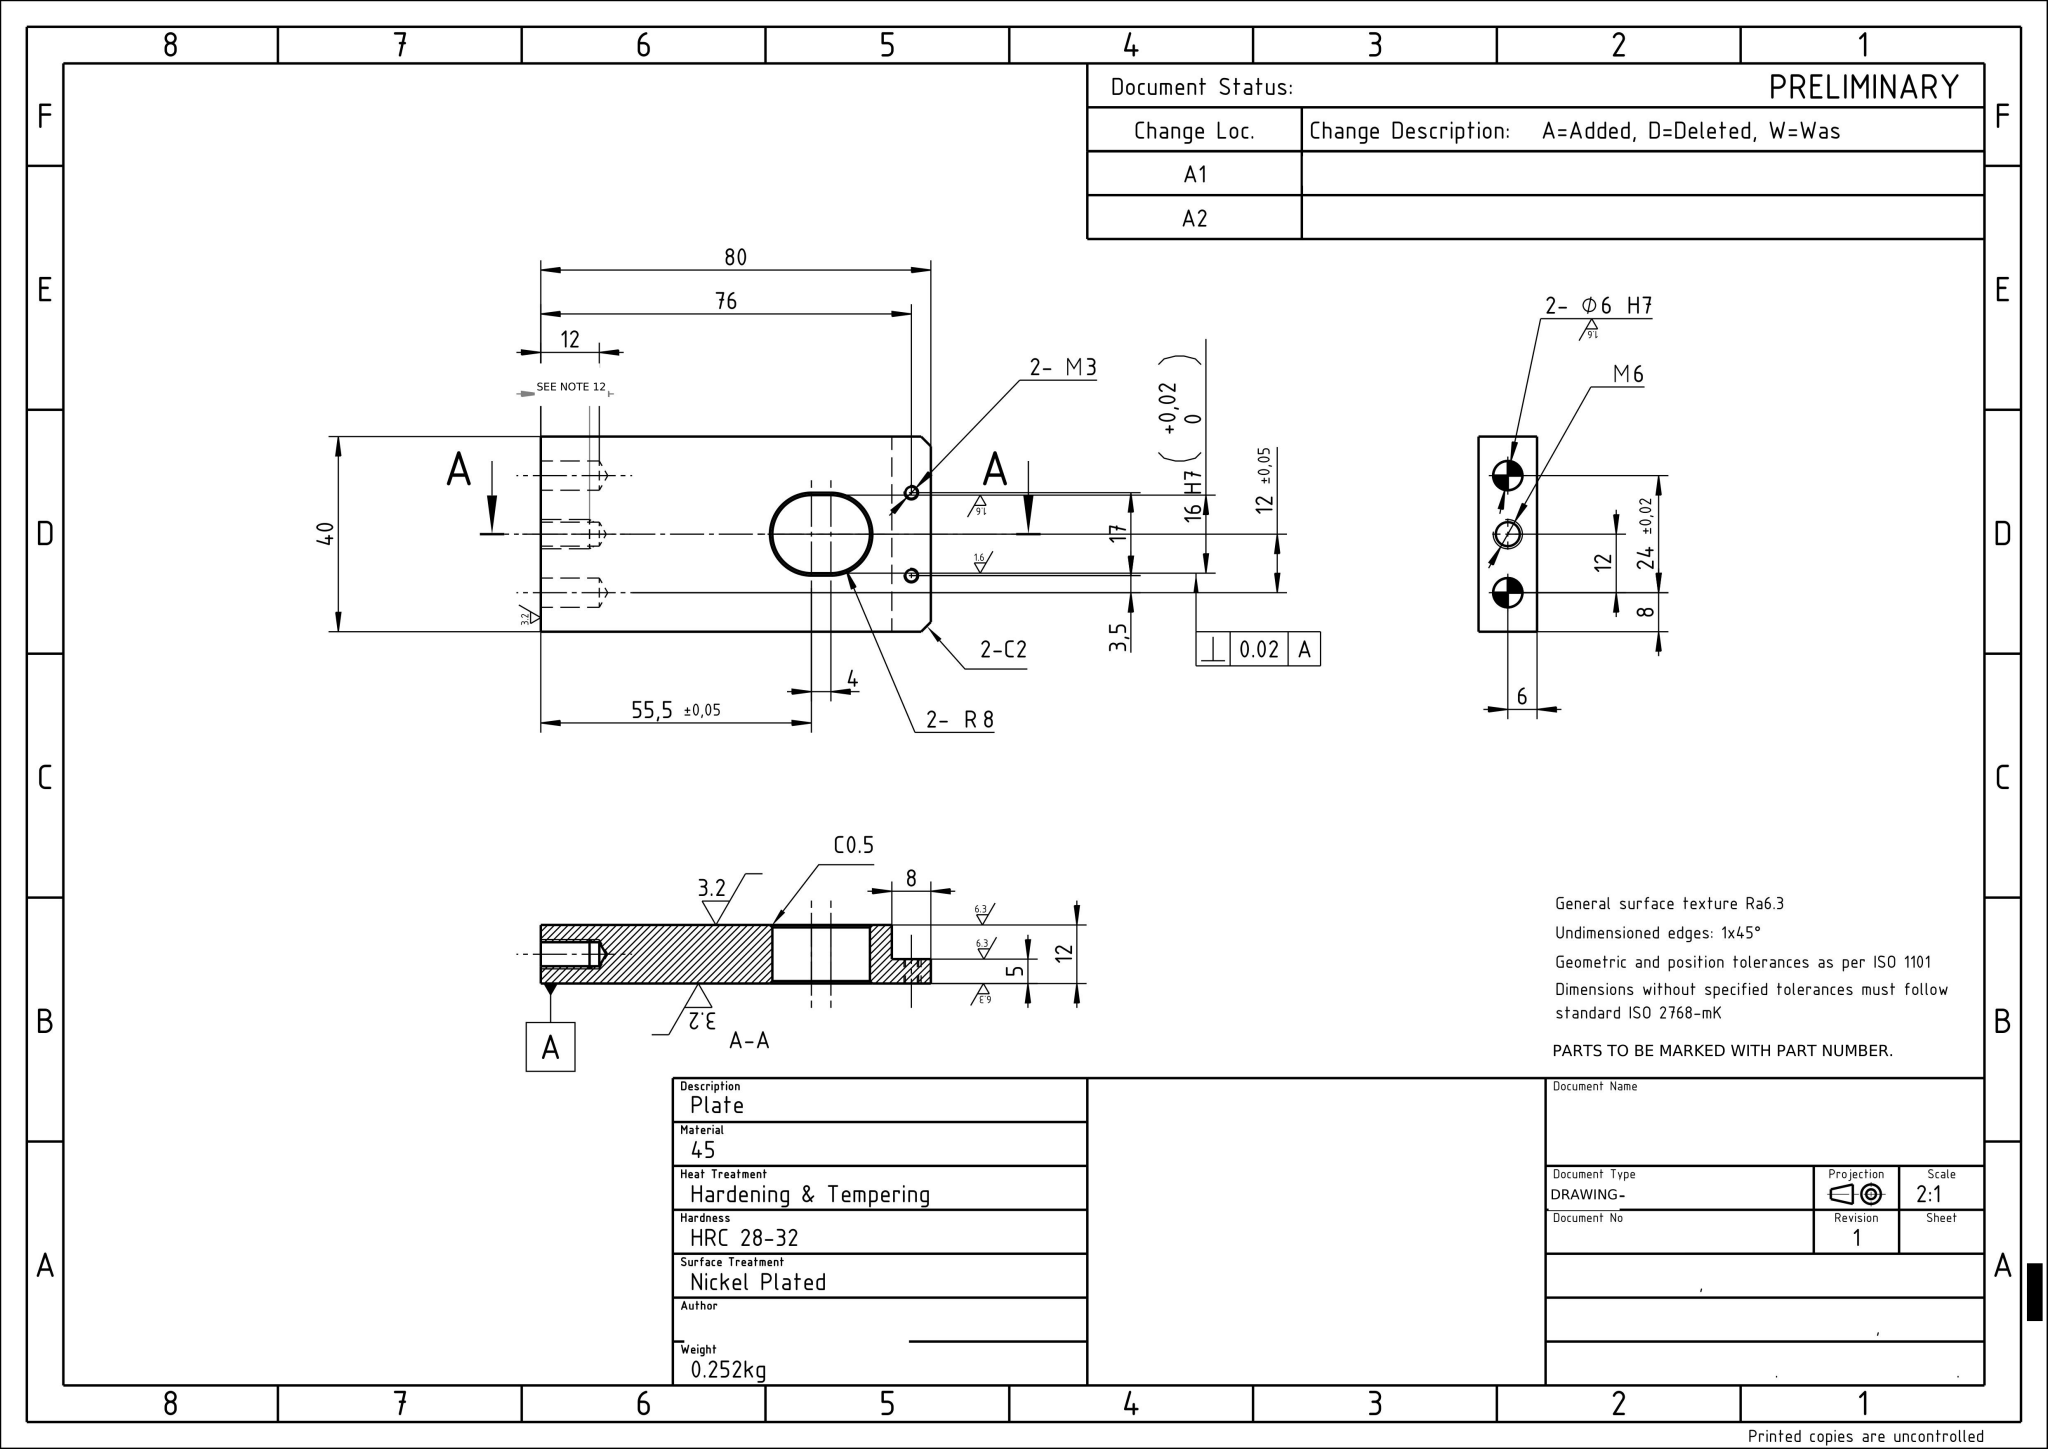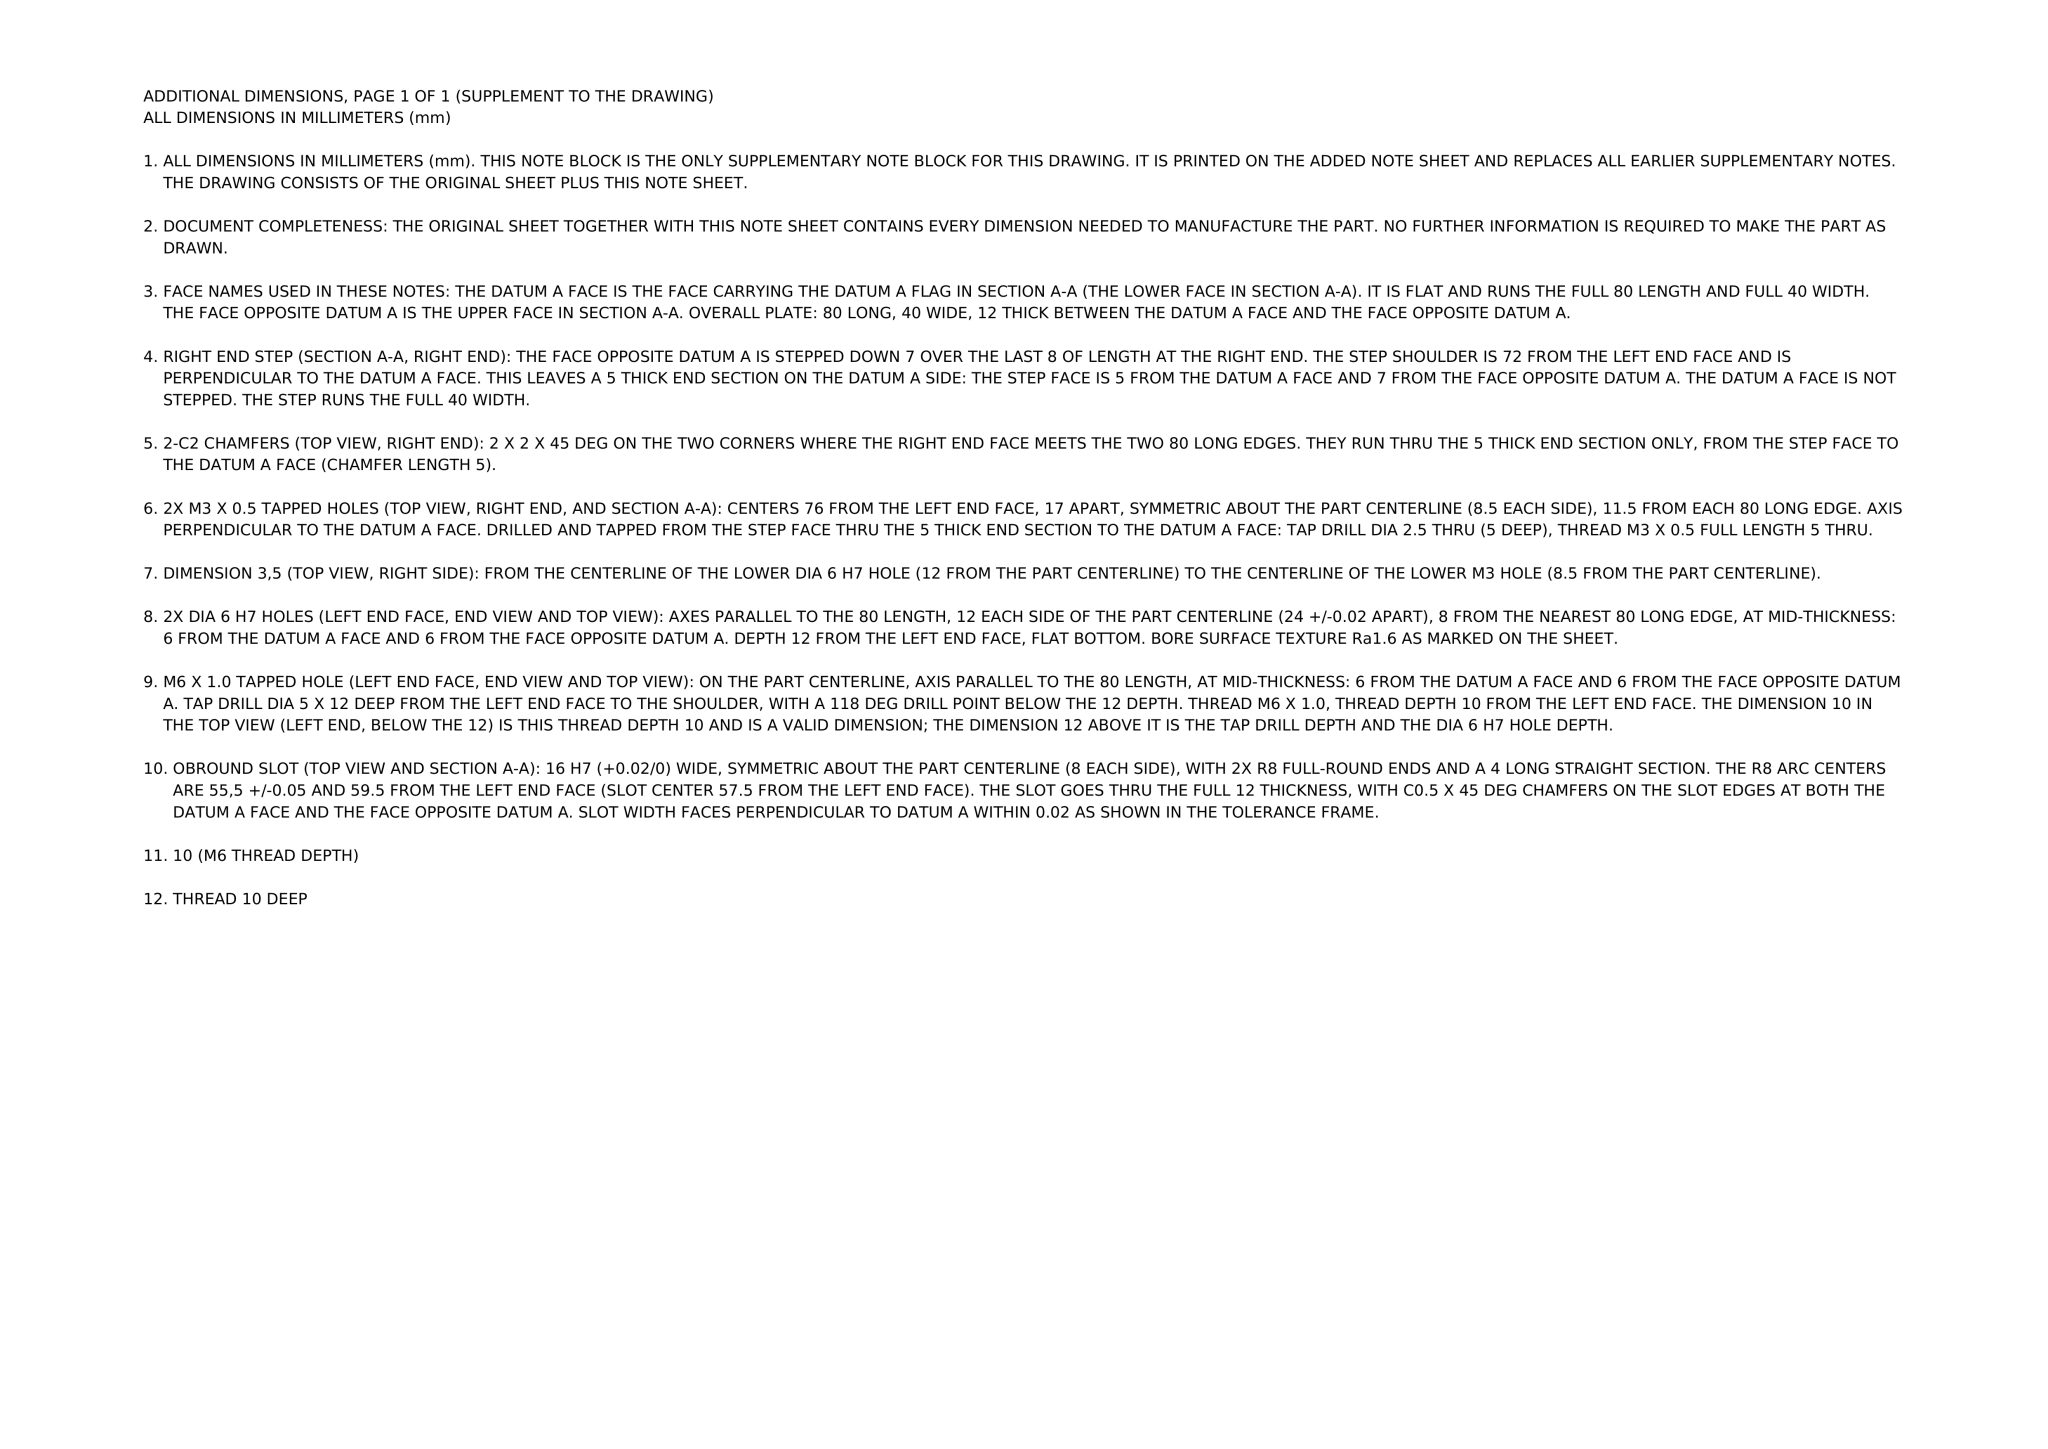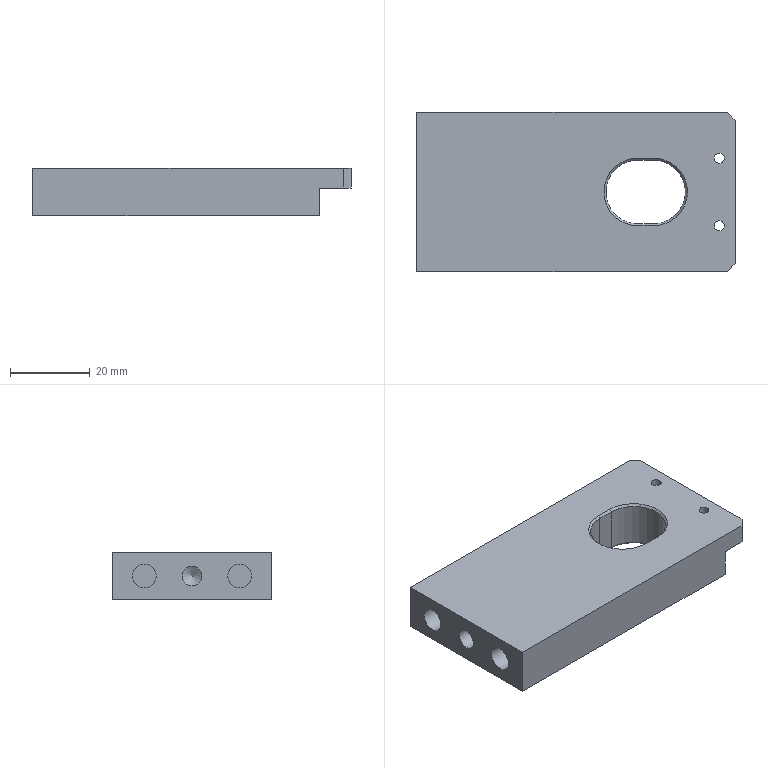Part | NX | mm | 1 solid | 30 faces | box 80 x 40 x 12 mm | volume 31971 mm3 | plane 18 | cylinder 7 | cone 5 | commonest cylinder face diameters 16 x2 2.5 x2 6 x2 5 x1
STEP:
#1=CARTESIAN_POINT('',(0.,0.,0.));
#2=DIRECTION('',(0.,0.,1.));
#3=DIRECTION('',(1.,0.,0.));
#4=AXIS2_PLACEMENT_3D('',#1,#2,#3);
#5=(LENGTH_UNIT()NAMED_UNIT(*)SI_UNIT(.MILLI.,.METRE.));
#6=UNCERTAINTY_MEASURE_WITH_UNIT(LENGTH_MEASURE(0.00002),#5,'','');
#7=(NAMED_UNIT(*)PLANE_ANGLE_UNIT()SI_UNIT($,.RADIAN.));
#8=PLANE_ANGLE_MEASURE_WITH_UNIT(PLANE_ANGLE_MEASURE(0.01745),#7);
#9=DIMENSIONAL_EXPONENTS(0.,0.,0.,0.,0.,0.,0.);
#10=(CONVERSION_BASED_UNIT('',#8)NAMED_UNIT(#9)PLANE_ANGLE_UNIT());
#11=(NAMED_UNIT(*)SI_UNIT($,.STERADIAN.)SOLID_ANGLE_UNIT());
#12=(GEOMETRIC_REPRESENTATION_CONTEXT(3)GLOBAL_UNCERTAINTY_ASSIGNED_CONTEXT((#6))GLOBAL_UNIT_ASSIGNED_CONTEXT((#5,#10,#11))REPRESENTATION_CONTEXT('',''));
#13=SHAPE_REPRESENTATION('',(#4),#12);
#14=CARTESIAN_POINT('',(34.75,8.5,12.));
#15=VERTEX_POINT('',#14);
#16=CARTESIAN_POINT('',(36.,8.5,12.));
#17=DIRECTION('',(0.,0.,-1.));
#18=DIRECTION('',(-1.,0.,0.));
#19=AXIS2_PLACEMENT_3D('',#16,#17,#18);
#20=CIRCLE('',#19,1.25);
#21=EDGE_CURVE('',#15,#15,#20,.T.);
#22=ORIENTED_EDGE('',*,*,#21,.T.);
#23=EDGE_LOOP('',(#22));
#24=FACE_BOUND('',#23,.T.);
#25=CARTESIAN_POINT('',(34.75,-8.5,12.));
#26=VERTEX_POINT('',#25);
#27=CARTESIAN_POINT('',(36.,-8.5,12.));
#28=DIRECTION('',(0.,0.,-1.));
#29=DIRECTION('',(-1.,0.,0.));
#30=AXIS2_PLACEMENT_3D('',#27,#28,#29);
#31=CIRCLE('',#30,1.25);
#32=EDGE_CURVE('',#26,#26,#31,.T.);
#33=ORIENTED_EDGE('',*,*,#32,.T.);
#34=EDGE_LOOP('',(#33));
#35=FACE_BOUND('',#34,.T.);
#36=CARTESIAN_POINT('',(19.5,-8.5,12.));
#37=VERTEX_POINT('',#36);
#38=CARTESIAN_POINT('',(15.5,-8.5,12.));
#39=VERTEX_POINT('',#38);
#40=CARTESIAN_POINT('',(0.,-8.5,12.));
#41=DIRECTION('',(-1.,0.,0.));
#42=VECTOR('',#41,1.);
#43=LINE('',#40,#42);
#44=EDGE_CURVE('',#37,#39,#43,.T.);
#45=ORIENTED_EDGE('',*,*,#44,.T.);
#46=CARTESIAN_POINT('',(15.5,8.5,12.));
#47=VERTEX_POINT('',#46);
#48=CARTESIAN_POINT('',(15.5,0.,12.));
#49=DIRECTION('',(0.,0.,-1.));
#50=DIRECTION('',(1.,0.,0.));
#51=AXIS2_PLACEMENT_3D('',#48,#49,#50);
#52=CIRCLE('',#51,8.5);
#53=EDGE_CURVE('',#39,#47,#52,.T.);
#54=ORIENTED_EDGE('',*,*,#53,.T.);
#55=CARTESIAN_POINT('',(19.5,8.5,12.));
#56=VERTEX_POINT('',#55);
#57=CARTESIAN_POINT('',(0.,8.5,12.));
#58=DIRECTION('',(1.,0.,0.));
#59=VECTOR('',#58,1.);
#60=LINE('',#57,#59);
#61=EDGE_CURVE('',#47,#56,#60,.T.);
#62=ORIENTED_EDGE('',*,*,#61,.T.);
#63=CARTESIAN_POINT('',(19.5,-0.,12.));
#64=DIRECTION('',(0.,0.,-1.));
#65=DIRECTION('',(1.,0.,0.));
#66=AXIS2_PLACEMENT_3D('',#63,#64,#65);
#67=CIRCLE('',#66,8.5);
#68=EDGE_CURVE('',#56,#37,#67,.T.);
#69=ORIENTED_EDGE('',*,*,#68,.T.);
#70=EDGE_LOOP('',(#45,#54,#62,#69));
#71=FACE_BOUND('',#70,.T.);
#72=CARTESIAN_POINT('',(40.,-18.,12.));
#73=VERTEX_POINT('',#72);
#74=CARTESIAN_POINT('',(40.,18.,12.));
#75=VERTEX_POINT('',#74);
#76=CARTESIAN_POINT('',(40.,-20.,12.));
#77=DIRECTION('',(-0.,1.,0.));
#78=VECTOR('',#77,1.);
#79=LINE('',#76,#78);
#80=EDGE_CURVE('',#73,#75,#79,.T.);
#81=ORIENTED_EDGE('',*,*,#80,.T.);
#82=CARTESIAN_POINT('',(38.,20.,12.));
#83=VERTEX_POINT('',#82);
#84=CARTESIAN_POINT('',(29.,29.,12.));
#85=DIRECTION('',(-0.7071,0.7071,0.));
#86=VECTOR('',#85,1.);
#87=LINE('',#84,#86);
#88=EDGE_CURVE('',#75,#83,#87,.T.);
#89=ORIENTED_EDGE('',*,*,#88,.T.);
#90=CARTESIAN_POINT('',(-40.,20.,12.));
#91=VERTEX_POINT('',#90);
#92=CARTESIAN_POINT('',(40.,20.,12.));
#93=DIRECTION('',(-1.,0.,0.));
#94=VECTOR('',#93,1.);
#95=LINE('',#92,#94);
#96=EDGE_CURVE('',#83,#91,#95,.T.);
#97=ORIENTED_EDGE('',*,*,#96,.T.);
#98=CARTESIAN_POINT('',(-40.,-20.,12.));
#99=VERTEX_POINT('',#98);
#100=CARTESIAN_POINT('',(-40.,20.,12.));
#101=DIRECTION('',(0.,-1.,0.));
#102=VECTOR('',#101,1.);
#103=LINE('',#100,#102);
#104=EDGE_CURVE('',#91,#99,#103,.T.);
#105=ORIENTED_EDGE('',*,*,#104,.T.);
#106=CARTESIAN_POINT('',(38.,-20.,12.));
#107=VERTEX_POINT('',#106);
#108=CARTESIAN_POINT('',(-40.,-20.,12.));
#109=DIRECTION('',(1.,0.,0.));
#110=VECTOR('',#109,1.);
#111=LINE('',#108,#110);
#112=EDGE_CURVE('',#99,#107,#111,.T.);
#113=ORIENTED_EDGE('',*,*,#112,.T.);
#114=CARTESIAN_POINT('',(29.,-29.,12.));
#115=DIRECTION('',(0.7071,0.7071,0.));
#116=VECTOR('',#115,1.);
#117=LINE('',#114,#116);
#118=EDGE_CURVE('',#107,#73,#117,.T.);
#119=ORIENTED_EDGE('',*,*,#118,.T.);
#120=EDGE_LOOP('',(#81,#89,#97,#105,#113,#119));
#121=FACE_BOUND('',#120,.T.);
#122=CARTESIAN_POINT('',(0.,0.,12.));
#123=DIRECTION('',(0.,0.,1.));
#124=DIRECTION('',(1.,0.,0.));
#125=AXIS2_PLACEMENT_3D('',#122,#123,#124);
#126=PLANE('',#125);
#127=ADVANCED_FACE('',(#24,#35,#71,#121),#126,.T.);
#128=CARTESIAN_POINT('',(19.5,8.5,0.));
#129=VERTEX_POINT('',#128);
#130=CARTESIAN_POINT('',(15.5,8.5,0.));
#131=VERTEX_POINT('',#130);
#132=CARTESIAN_POINT('',(15.5,8.5,0.));
#133=DIRECTION('',(-1.,0.,0.));
#134=VECTOR('',#133,1.);
#135=LINE('',#132,#134);
#136=EDGE_CURVE('',#129,#131,#135,.T.);
#137=ORIENTED_EDGE('',*,*,#136,.T.);
#138=CARTESIAN_POINT('',(15.5,-8.5,0.));
#139=VERTEX_POINT('',#138);
#140=CARTESIAN_POINT('',(15.5,0.,0.));
#141=DIRECTION('',(0.,0.,1.));
#142=DIRECTION('',(1.,0.,0.));
#143=AXIS2_PLACEMENT_3D('',#140,#141,#142);
#144=CIRCLE('',#143,8.5);
#145=EDGE_CURVE('',#131,#139,#144,.T.);
#146=ORIENTED_EDGE('',*,*,#145,.T.);
#147=CARTESIAN_POINT('',(19.5,-8.5,0.));
#148=VERTEX_POINT('',#147);
#149=CARTESIAN_POINT('',(19.5,-8.5,0.));
#150=DIRECTION('',(1.,0.,0.));
#151=VECTOR('',#150,1.);
#152=LINE('',#149,#151);
#153=EDGE_CURVE('',#139,#148,#152,.T.);
#154=ORIENTED_EDGE('',*,*,#153,.T.);
#155=CARTESIAN_POINT('',(19.5,-0.,0.));
#156=DIRECTION('',(0.,0.,1.));
#157=DIRECTION('',(1.,0.,0.));
#158=AXIS2_PLACEMENT_3D('',#155,#156,#157);
#159=CIRCLE('',#158,8.5);
#160=EDGE_CURVE('',#148,#129,#159,.T.);
#161=ORIENTED_EDGE('',*,*,#160,.T.);
#162=EDGE_LOOP('',(#137,#146,#154,#161));
#163=FACE_BOUND('',#162,.T.);
#164=CARTESIAN_POINT('',(32.,20.,0.));
#165=VERTEX_POINT('',#164);
#166=CARTESIAN_POINT('',(-40.,20.,0.));
#167=VERTEX_POINT('',#166);
#168=CARTESIAN_POINT('',(40.,20.,0.));
#169=DIRECTION('',(-1.,0.,0.));
#170=VECTOR('',#169,1.);
#171=LINE('',#168,#170);
#172=EDGE_CURVE('',#165,#167,#171,.T.);
#173=ORIENTED_EDGE('',*,*,#172,.F.);
#174=CARTESIAN_POINT('',(32.,-20.,0.));
#175=VERTEX_POINT('',#174);
#176=CARTESIAN_POINT('',(32.,20.,0.));
#177=DIRECTION('',(0.,-1.,0.));
#178=VECTOR('',#177,1.);
#179=LINE('',#176,#178);
#180=EDGE_CURVE('',#165,#175,#179,.T.);
#181=ORIENTED_EDGE('',*,*,#180,.T.);
#182=CARTESIAN_POINT('',(-40.,-20.,0.));
#183=VERTEX_POINT('',#182);
#184=CARTESIAN_POINT('',(-40.,-20.,0.));
#185=DIRECTION('',(1.,0.,0.));
#186=VECTOR('',#185,1.);
#187=LINE('',#184,#186);
#188=EDGE_CURVE('',#183,#175,#187,.T.);
#189=ORIENTED_EDGE('',*,*,#188,.F.);
#190=CARTESIAN_POINT('',(-40.,20.,0.));
#191=DIRECTION('',(0.,-1.,0.));
#192=VECTOR('',#191,1.);
#193=LINE('',#190,#192);
#194=EDGE_CURVE('',#167,#183,#193,.T.);
#195=ORIENTED_EDGE('',*,*,#194,.F.);
#196=EDGE_LOOP('',(#173,#181,#189,#195));
#197=FACE_BOUND('',#196,.T.);
#198=CARTESIAN_POINT('',(0.,0.,0.));
#199=DIRECTION('',(0.,0.,1.));
#200=DIRECTION('',(1.,0.,0.));
#201=AXIS2_PLACEMENT_3D('',#198,#199,#200);
#202=PLANE('',#201);
#203=ADVANCED_FACE('',(#163,#197),#202,.F.);
#204=CARTESIAN_POINT('',(38.,-20.,7.));
#205=VERTEX_POINT('',#204);
#206=CARTESIAN_POINT('',(32.,-20.,7.));
#207=VERTEX_POINT('',#206);
#208=CARTESIAN_POINT('',(40.,-20.,7.));
#209=DIRECTION('',(-1.,-0.,0.));
#210=VECTOR('',#209,1.);
#211=LINE('',#208,#210);
#212=EDGE_CURVE('',#205,#207,#211,.T.);
#213=ORIENTED_EDGE('',*,*,#212,.F.);
#214=CARTESIAN_POINT('',(38.,-20.,12.));
#215=DIRECTION('',(0.,0.,1.));
#216=VECTOR('',#215,1.);
#217=LINE('',#214,#216);
#218=EDGE_CURVE('',#205,#107,#217,.T.);
#219=ORIENTED_EDGE('',*,*,#218,.T.);
#220=ORIENTED_EDGE('',*,*,#112,.F.);
#221=CARTESIAN_POINT('',(-40.,-20.,12.));
#222=DIRECTION('',(0.,0.,-1.));
#223=VECTOR('',#222,1.);
#224=LINE('',#221,#223);
#225=EDGE_CURVE('',#99,#183,#224,.T.);
#226=ORIENTED_EDGE('',*,*,#225,.T.);
#227=ORIENTED_EDGE('',*,*,#188,.T.);
#228=CARTESIAN_POINT('',(32.,-20.,0.));
#229=DIRECTION('',(0.,0.,1.));
#230=VECTOR('',#229,1.);
#231=LINE('',#228,#230);
#232=EDGE_CURVE('',#175,#207,#231,.T.);
#233=ORIENTED_EDGE('',*,*,#232,.T.);
#234=EDGE_LOOP('',(#213,#219,#220,#226,#227,#233));
#235=FACE_OUTER_BOUND('',#234,.T.);
#236=CARTESIAN_POINT('',(-40.,-20.,12.));
#237=DIRECTION('',(0.,1.,0.));
#238=DIRECTION('',(0.,0.,1.));
#239=AXIS2_PLACEMENT_3D('',#236,#237,#238);
#240=PLANE('',#239);
#241=ADVANCED_FACE('',(#235),#240,.F.);
#242=CARTESIAN_POINT('',(40.,18.,7.));
#243=VERTEX_POINT('',#242);
#244=CARTESIAN_POINT('',(40.,-18.,7.));
#245=VERTEX_POINT('',#244);
#246=CARTESIAN_POINT('',(40.,20.,7.));
#247=DIRECTION('',(0.,-1.,0.));
#248=VECTOR('',#247,1.);
#249=LINE('',#246,#248);
#250=EDGE_CURVE('',#243,#245,#249,.T.);
#251=ORIENTED_EDGE('',*,*,#250,.F.);
#252=CARTESIAN_POINT('',(40.,18.,12.));
#253=DIRECTION('',(0.,0.,1.));
#254=VECTOR('',#253,1.);
#255=LINE('',#252,#254);
#256=EDGE_CURVE('',#243,#75,#255,.T.);
#257=ORIENTED_EDGE('',*,*,#256,.T.);
#258=ORIENTED_EDGE('',*,*,#80,.F.);
#259=CARTESIAN_POINT('',(40.,-18.,12.));
#260=DIRECTION('',(0.,0.,-1.));
#261=VECTOR('',#260,1.);
#262=LINE('',#259,#261);
#263=EDGE_CURVE('',#73,#245,#262,.T.);
#264=ORIENTED_EDGE('',*,*,#263,.T.);
#265=EDGE_LOOP('',(#251,#257,#258,#264));
#266=FACE_OUTER_BOUND('',#265,.T.);
#267=CARTESIAN_POINT('',(40.,-20.,12.));
#268=DIRECTION('',(-1.,-0.,0.));
#269=DIRECTION('',(0.,-1.,0.));
#270=AXIS2_PLACEMENT_3D('',#267,#268,#269);
#271=PLANE('',#270);
#272=ADVANCED_FACE('',(#266),#271,.F.);
#273=ORIENTED_EDGE('',*,*,#96,.F.);
#274=CARTESIAN_POINT('',(38.,20.,7.));
#275=VERTEX_POINT('',#274);
#276=CARTESIAN_POINT('',(38.,20.,12.));
#277=DIRECTION('',(0.,0.,-1.));
#278=VECTOR('',#277,1.);
#279=LINE('',#276,#278);
#280=EDGE_CURVE('',#83,#275,#279,.T.);
#281=ORIENTED_EDGE('',*,*,#280,.T.);
#282=CARTESIAN_POINT('',(32.,20.,7.));
#283=VERTEX_POINT('',#282);
#284=CARTESIAN_POINT('',(40.,20.,7.));
#285=DIRECTION('',(-1.,-0.,0.));
#286=VECTOR('',#285,1.);
#287=LINE('',#284,#286);
#288=EDGE_CURVE('',#275,#283,#287,.T.);
#289=ORIENTED_EDGE('',*,*,#288,.T.);
#290=CARTESIAN_POINT('',(32.,20.,0.));
#291=DIRECTION('',(0.,0.,1.));
#292=VECTOR('',#291,1.);
#293=LINE('',#290,#292);
#294=EDGE_CURVE('',#165,#283,#293,.T.);
#295=ORIENTED_EDGE('',*,*,#294,.F.);
#296=ORIENTED_EDGE('',*,*,#172,.T.);
#297=CARTESIAN_POINT('',(-40.,20.,12.));
#298=DIRECTION('',(0.,0.,-1.));
#299=VECTOR('',#298,1.);
#300=LINE('',#297,#299);
#301=EDGE_CURVE('',#91,#167,#300,.T.);
#302=ORIENTED_EDGE('',*,*,#301,.F.);
#303=EDGE_LOOP('',(#273,#281,#289,#295,#296,#302));
#304=FACE_OUTER_BOUND('',#303,.T.);
#305=CARTESIAN_POINT('',(40.,20.,12.));
#306=DIRECTION('',(0.,-1.,0.));
#307=DIRECTION('',(0.,0.,-1.));
#308=AXIS2_PLACEMENT_3D('',#305,#306,#307);
#309=PLANE('',#308);
#310=ADVANCED_FACE('',(#304),#309,.F.);
#311=CARTESIAN_POINT('',(-40.,15.,6.));
#312=VERTEX_POINT('',#311);
#313=CARTESIAN_POINT('',(-40.,12.,6.));
#314=DIRECTION('',(1.,0.,0.));
#315=DIRECTION('',(-0.,1.,0.));
#316=AXIS2_PLACEMENT_3D('',#313,#314,#315);
#317=CIRCLE('',#316,3.);
#318=EDGE_CURVE('',#312,#312,#317,.T.);
#319=ORIENTED_EDGE('',*,*,#318,.T.);
#320=EDGE_LOOP('',(#319));
#321=FACE_BOUND('',#320,.T.);
#322=CARTESIAN_POINT('',(-40.,-9.,6.));
#323=VERTEX_POINT('',#322);
#324=CARTESIAN_POINT('',(-40.,-12.,6.));
#325=DIRECTION('',(1.,0.,0.));
#326=DIRECTION('',(-0.,1.,0.));
#327=AXIS2_PLACEMENT_3D('',#324,#325,#326);
#328=CIRCLE('',#327,3.);
#329=EDGE_CURVE('',#323,#323,#328,.T.);
#330=ORIENTED_EDGE('',*,*,#329,.T.);
#331=EDGE_LOOP('',(#330));
#332=FACE_BOUND('',#331,.T.);
#333=CARTESIAN_POINT('',(-40.,2.5,6.));
#334=VERTEX_POINT('',#333);
#335=CARTESIAN_POINT('',(-40.,-0.,6.));
#336=DIRECTION('',(1.,0.,0.));
#337=DIRECTION('',(0.,1.,0.));
#338=AXIS2_PLACEMENT_3D('',#335,#336,#337);
#339=CIRCLE('',#338,2.5);
#340=EDGE_CURVE('',#334,#334,#339,.T.);
#341=ORIENTED_EDGE('',*,*,#340,.T.);
#342=EDGE_LOOP('',(#341));
#343=FACE_BOUND('',#342,.T.);
#344=ORIENTED_EDGE('',*,*,#194,.T.);
#345=ORIENTED_EDGE('',*,*,#225,.F.);
#346=ORIENTED_EDGE('',*,*,#104,.F.);
#347=ORIENTED_EDGE('',*,*,#301,.T.);
#348=EDGE_LOOP('',(#344,#345,#346,#347));
#349=FACE_BOUND('',#348,.T.);
#350=CARTESIAN_POINT('',(-40.,20.,12.));
#351=DIRECTION('',(1.,0.,0.));
#352=DIRECTION('',(-0.,1.,0.));
#353=AXIS2_PLACEMENT_3D('',#350,#351,#352);
#354=PLANE('',#353);
#355=ADVANCED_FACE('',(#321,#332,#343,#349),#354,.F.);
#356=CARTESIAN_POINT('',(34.75,8.5,7.));
#357=VERTEX_POINT('',#356);
#358=CARTESIAN_POINT('',(36.,8.5,7.));
#359=DIRECTION('',(0.,0.,1.));
#360=DIRECTION('',(-1.,0.,0.));
#361=AXIS2_PLACEMENT_3D('',#358,#359,#360);
#362=CIRCLE('',#361,1.25);
#363=EDGE_CURVE('',#357,#357,#362,.T.);
#364=ORIENTED_EDGE('',*,*,#363,.T.);
#365=EDGE_LOOP('',(#364));
#366=FACE_BOUND('',#365,.T.);
#367=CARTESIAN_POINT('',(34.75,-8.5,7.));
#368=VERTEX_POINT('',#367);
#369=CARTESIAN_POINT('',(36.,-8.5,7.));
#370=DIRECTION('',(0.,0.,1.));
#371=DIRECTION('',(-1.,0.,0.));
#372=AXIS2_PLACEMENT_3D('',#369,#370,#371);
#373=CIRCLE('',#372,1.25);
#374=EDGE_CURVE('',#368,#368,#373,.T.);
#375=ORIENTED_EDGE('',*,*,#374,.T.);
#376=EDGE_LOOP('',(#375));
#377=FACE_BOUND('',#376,.T.);
#378=ORIENTED_EDGE('',*,*,#288,.F.);
#379=CARTESIAN_POINT('',(38.,20.,7.));
#380=DIRECTION('',(0.7071,-0.7071,0.));
#381=VECTOR('',#380,1.);
#382=LINE('',#379,#381);
#383=EDGE_CURVE('',#275,#243,#382,.T.);
#384=ORIENTED_EDGE('',*,*,#383,.T.);
#385=ORIENTED_EDGE('',*,*,#250,.T.);
#386=CARTESIAN_POINT('',(40.,-18.,7.));
#387=DIRECTION('',(-0.7071,-0.7071,0.));
#388=VECTOR('',#387,1.);
#389=LINE('',#386,#388);
#390=EDGE_CURVE('',#245,#205,#389,.T.);
#391=ORIENTED_EDGE('',*,*,#390,.T.);
#392=ORIENTED_EDGE('',*,*,#212,.T.);
#393=CARTESIAN_POINT('',(32.,20.,7.));
#394=DIRECTION('',(-0.,1.,0.));
#395=VECTOR('',#394,1.);
#396=LINE('',#393,#395);
#397=EDGE_CURVE('',#207,#283,#396,.T.);
#398=ORIENTED_EDGE('',*,*,#397,.T.);
#399=EDGE_LOOP('',(#378,#384,#385,#391,#392,#398));
#400=FACE_BOUND('',#399,.T.);
#401=CARTESIAN_POINT('',(40.,20.,7.));
#402=DIRECTION('',(0.,0.,-1.));
#403=DIRECTION('',(0.,-1.,0.));
#404=AXIS2_PLACEMENT_3D('',#401,#402,#403);
#405=PLANE('',#404);
#406=ADVANCED_FACE('',(#366,#377,#400),#405,.T.);
#407=ORIENTED_EDGE('',*,*,#397,.F.);
#408=ORIENTED_EDGE('',*,*,#232,.F.);
#409=ORIENTED_EDGE('',*,*,#180,.F.);
#410=ORIENTED_EDGE('',*,*,#294,.T.);
#411=EDGE_LOOP('',(#407,#408,#409,#410));
#412=FACE_OUTER_BOUND('',#411,.T.);
#413=CARTESIAN_POINT('',(32.,20.,0.));
#414=DIRECTION('',(-1.,-0.,0.));
#415=DIRECTION('',(0.,-1.,0.));
#416=AXIS2_PLACEMENT_3D('',#413,#414,#415);
#417=PLANE('',#416);
#418=ADVANCED_FACE('',(#412),#417,.F.);
#419=CARTESIAN_POINT('',(15.5,-8.,0.5));
#420=VERTEX_POINT('',#419);
#421=CARTESIAN_POINT('',(15.5,-8.,11.5));
#422=VERTEX_POINT('',#421);
#423=CARTESIAN_POINT('',(15.5,-8.,55000.));
#424=DIRECTION('',(0.,0.,1.));
#425=VECTOR('',#424,1.);
#426=LINE('',#423,#425);
#427=EDGE_CURVE('',#420,#422,#426,.T.);
#428=ORIENTED_EDGE('',*,*,#427,.F.);
#429=CARTESIAN_POINT('',(15.5,8.,0.5));
#430=VERTEX_POINT('',#429);
#431=CARTESIAN_POINT('',(15.5,0.,0.5));
#432=DIRECTION('',(0.,0.,-1.));
#433=DIRECTION('',(1.,0.,0.));
#434=AXIS2_PLACEMENT_3D('',#431,#432,#433);
#435=CIRCLE('',#434,8.);
#436=EDGE_CURVE('',#420,#430,#435,.T.);
#437=ORIENTED_EDGE('',*,*,#436,.T.);
#438=CARTESIAN_POINT('',(15.5,8.,11.5));
#439=VERTEX_POINT('',#438);
#440=CARTESIAN_POINT('',(15.5,8.,55000.));
#441=DIRECTION('',(0.,0.,1.));
#442=VECTOR('',#441,1.);
#443=LINE('',#440,#442);
#444=EDGE_CURVE('',#430,#439,#443,.T.);
#445=ORIENTED_EDGE('',*,*,#444,.T.);
#446=CARTESIAN_POINT('',(15.5,0.,11.5));
#447=DIRECTION('',(0.,0.,1.));
#448=DIRECTION('',(1.,0.,0.));
#449=AXIS2_PLACEMENT_3D('',#446,#447,#448);
#450=CIRCLE('',#449,8.);
#451=EDGE_CURVE('',#439,#422,#450,.T.);
#452=ORIENTED_EDGE('',*,*,#451,.T.);
#453=EDGE_LOOP('',(#428,#437,#445,#452));
#454=FACE_OUTER_BOUND('',#453,.T.);
#455=CARTESIAN_POINT('',(15.5,0.,55000.));
#456=DIRECTION('',(0.,0.,-1.));
#457=DIRECTION('',(-1.,0.,0.));
#458=AXIS2_PLACEMENT_3D('',#455,#456,#457);
#459=CYLINDRICAL_SURFACE('',#458,8.);
#460=ADVANCED_FACE('',(#454),#459,.F.);
#461=CARTESIAN_POINT('',(19.5,-8.,0.5));
#462=VERTEX_POINT('',#461);
#463=CARTESIAN_POINT('',(19.5,-8.,11.5));
#464=VERTEX_POINT('',#463);
#465=CARTESIAN_POINT('',(19.5,-8.,55000.));
#466=DIRECTION('',(0.,0.,1.));
#467=VECTOR('',#466,1.);
#468=LINE('',#465,#467);
#469=EDGE_CURVE('',#462,#464,#468,.T.);
#470=ORIENTED_EDGE('',*,*,#469,.F.);
#471=CARTESIAN_POINT('',(15.5,-8.,0.5));
#472=DIRECTION('',(-1.,0.,0.));
#473=VECTOR('',#472,1.);
#474=LINE('',#471,#473);
#475=EDGE_CURVE('',#462,#420,#474,.T.);
#476=ORIENTED_EDGE('',*,*,#475,.T.);
#477=ORIENTED_EDGE('',*,*,#427,.T.);
#478=CARTESIAN_POINT('',(15.5,-8.,11.5));
#479=DIRECTION('',(1.,0.,0.));
#480=VECTOR('',#479,1.);
#481=LINE('',#478,#480);
#482=EDGE_CURVE('',#422,#464,#481,.T.);
#483=ORIENTED_EDGE('',*,*,#482,.T.);
#484=EDGE_LOOP('',(#470,#476,#477,#483));
#485=FACE_OUTER_BOUND('',#484,.T.);
#486=CARTESIAN_POINT('',(15.5,-8.,55000.));
#487=DIRECTION('',(0.,1.,0.));
#488=DIRECTION('',(0.,0.,1.));
#489=AXIS2_PLACEMENT_3D('',#486,#487,#488);
#490=PLANE('',#489);
#491=ADVANCED_FACE('',(#485),#490,.T.);
#492=CARTESIAN_POINT('',(19.5,8.,0.5));
#493=VERTEX_POINT('',#492);
#494=CARTESIAN_POINT('',(19.5,8.,11.5));
#495=VERTEX_POINT('',#494);
#496=CARTESIAN_POINT('',(19.5,8.,55000.));
#497=DIRECTION('',(0.,0.,1.));
#498=VECTOR('',#497,1.);
#499=LINE('',#496,#498);
#500=EDGE_CURVE('',#493,#495,#499,.T.);
#501=ORIENTED_EDGE('',*,*,#500,.F.);
#502=CARTESIAN_POINT('',(19.5,-0.,0.5));
#503=DIRECTION('',(0.,0.,-1.));
#504=DIRECTION('',(1.,0.,0.));
#505=AXIS2_PLACEMENT_3D('',#502,#503,#504);
#506=CIRCLE('',#505,8.);
#507=EDGE_CURVE('',#493,#462,#506,.T.);
#508=ORIENTED_EDGE('',*,*,#507,.T.);
#509=ORIENTED_EDGE('',*,*,#469,.T.);
#510=CARTESIAN_POINT('',(19.5,-0.,11.5));
#511=DIRECTION('',(0.,0.,1.));
#512=DIRECTION('',(1.,0.,0.));
#513=AXIS2_PLACEMENT_3D('',#510,#511,#512);
#514=CIRCLE('',#513,8.);
#515=EDGE_CURVE('',#464,#495,#514,.T.);
#516=ORIENTED_EDGE('',*,*,#515,.T.);
#517=EDGE_LOOP('',(#501,#508,#509,#516));
#518=FACE_OUTER_BOUND('',#517,.T.);
#519=CARTESIAN_POINT('',(19.5,-0.,55000.));
#520=DIRECTION('',(0.,0.,-1.));
#521=DIRECTION('',(-1.,0.,0.));
#522=AXIS2_PLACEMENT_3D('',#519,#520,#521);
#523=CYLINDRICAL_SURFACE('',#522,8.);
#524=ADVANCED_FACE('',(#518),#523,.F.);
#525=ORIENTED_EDGE('',*,*,#444,.F.);
#526=CARTESIAN_POINT('',(19.5,8.,0.5));
#527=DIRECTION('',(1.,0.,0.));
#528=VECTOR('',#527,1.);
#529=LINE('',#526,#528);
#530=EDGE_CURVE('',#430,#493,#529,.T.);
#531=ORIENTED_EDGE('',*,*,#530,.T.);
#532=ORIENTED_EDGE('',*,*,#500,.T.);
#533=CARTESIAN_POINT('',(19.5,8.,11.5));
#534=DIRECTION('',(-1.,0.,0.));
#535=VECTOR('',#534,1.);
#536=LINE('',#533,#535);
#537=EDGE_CURVE('',#495,#439,#536,.T.);
#538=ORIENTED_EDGE('',*,*,#537,.T.);
#539=EDGE_LOOP('',(#525,#531,#532,#538));
#540=FACE_OUTER_BOUND('',#539,.T.);
#541=CARTESIAN_POINT('',(19.5,8.,55000.));
#542=DIRECTION('',(0.,-1.,0.));
#543=DIRECTION('',(0.,0.,-1.));
#544=AXIS2_PLACEMENT_3D('',#541,#542,#543);
#545=PLANE('',#544);
#546=ADVANCED_FACE('',(#540),#545,.T.);
#547=ORIENTED_EDGE('',*,*,#88,.F.);
#548=ORIENTED_EDGE('',*,*,#256,.F.);
#549=ORIENTED_EDGE('',*,*,#383,.F.);
#550=ORIENTED_EDGE('',*,*,#280,.F.);
#551=EDGE_LOOP('',(#547,#548,#549,#550));
#552=FACE_OUTER_BOUND('',#551,.T.);
#553=CARTESIAN_POINT('',(38.,20.,12.));
#554=DIRECTION('',(-0.7071,-0.7071,0.));
#555=DIRECTION('',(0.,0.,-1.));
#556=AXIS2_PLACEMENT_3D('',#553,#554,#555);
#557=PLANE('',#556);
#558=ADVANCED_FACE('',(#552),#557,.F.);
#559=ORIENTED_EDGE('',*,*,#118,.F.);
#560=ORIENTED_EDGE('',*,*,#218,.F.);
#561=ORIENTED_EDGE('',*,*,#390,.F.);
#562=ORIENTED_EDGE('',*,*,#263,.F.);
#563=EDGE_LOOP('',(#559,#560,#561,#562));
#564=FACE_OUTER_BOUND('',#563,.T.);
#565=CARTESIAN_POINT('',(40.,-18.,12.));
#566=DIRECTION('',(-0.7071,0.7071,0.));
#567=DIRECTION('',(0.,0.,-1.));
#568=AXIS2_PLACEMENT_3D('',#565,#566,#567);
#569=PLANE('',#568);
#570=ADVANCED_FACE('',(#564),#569,.F.);
#571=CARTESIAN_POINT('',(19.5,-8.,0.5));
#572=DIRECTION('',(0.,-0.7071,-0.7071));
#573=VECTOR('',#572,1.);
#574=LINE('',#571,#573);
#575=EDGE_CURVE('',#462,#148,#574,.T.);
#576=ORIENTED_EDGE('',*,*,#575,.F.);
#577=ORIENTED_EDGE('',*,*,#507,.F.);
#578=CARTESIAN_POINT('',(19.5,8.5,0.));
#579=DIRECTION('',(0.,-0.7071,0.7071));
#580=VECTOR('',#579,1.);
#581=LINE('',#578,#580);
#582=EDGE_CURVE('',#129,#493,#581,.T.);
#583=ORIENTED_EDGE('',*,*,#582,.F.);
#584=ORIENTED_EDGE('',*,*,#160,.F.);
#585=EDGE_LOOP('',(#576,#577,#583,#584));
#586=FACE_OUTER_BOUND('',#585,.T.);
#587=CARTESIAN_POINT('',(19.5,-0.,0.));
#588=DIRECTION('',(0.,0.,-1.));
#589=DIRECTION('',(-1.,0.,0.));
#590=AXIS2_PLACEMENT_3D('',#587,#588,#589);
#591=CONICAL_SURFACE('',#590,8.5,45.);
#592=ADVANCED_FACE('',(#586),#591,.F.);
#593=ORIENTED_EDGE('',*,*,#582,.T.);
#594=ORIENTED_EDGE('',*,*,#530,.F.);
#595=CARTESIAN_POINT('',(15.5,8.5,0.));
#596=DIRECTION('',(0.,-0.7071,0.7071));
#597=VECTOR('',#596,1.);
#598=LINE('',#595,#597);
#599=EDGE_CURVE('',#131,#430,#598,.T.);
#600=ORIENTED_EDGE('',*,*,#599,.F.);
#601=ORIENTED_EDGE('',*,*,#136,.F.);
#602=EDGE_LOOP('',(#593,#594,#600,#601));
#603=FACE_OUTER_BOUND('',#602,.T.);
#604=CARTESIAN_POINT('',(0.,8.5,0.));
#605=DIRECTION('',(0.,-0.7071,-0.7071));
#606=DIRECTION('',(1.,0.,0.));
#607=AXIS2_PLACEMENT_3D('',#604,#605,#606);
#608=PLANE('',#607);
#609=ADVANCED_FACE('',(#603),#608,.T.);
#610=ORIENTED_EDGE('',*,*,#575,.T.);
#611=ORIENTED_EDGE('',*,*,#153,.F.);
#612=CARTESIAN_POINT('',(15.5,-8.,0.5));
#613=DIRECTION('',(0.,-0.7071,-0.7071));
#614=VECTOR('',#613,1.);
#615=LINE('',#612,#614);
#616=EDGE_CURVE('',#420,#139,#615,.T.);
#617=ORIENTED_EDGE('',*,*,#616,.F.);
#618=ORIENTED_EDGE('',*,*,#475,.F.);
#619=EDGE_LOOP('',(#610,#611,#617,#618));
#620=FACE_OUTER_BOUND('',#619,.T.);
#621=CARTESIAN_POINT('',(0.,-8.5,0.));
#622=DIRECTION('',(0.,0.7071,-0.7071));
#623=DIRECTION('',(-1.,0.,0.));
#624=AXIS2_PLACEMENT_3D('',#621,#622,#623);
#625=PLANE('',#624);
#626=ADVANCED_FACE('',(#620),#625,.T.);
#627=ORIENTED_EDGE('',*,*,#599,.T.);
#628=ORIENTED_EDGE('',*,*,#436,.F.);
#629=ORIENTED_EDGE('',*,*,#616,.T.);
#630=ORIENTED_EDGE('',*,*,#145,.F.);
#631=EDGE_LOOP('',(#627,#628,#629,#630));
#632=FACE_OUTER_BOUND('',#631,.T.);
#633=CARTESIAN_POINT('',(15.5,0.,0.));
#634=DIRECTION('',(0.,0.,-1.));
#635=DIRECTION('',(-1.,0.,0.));
#636=AXIS2_PLACEMENT_3D('',#633,#634,#635);
#637=CONICAL_SURFACE('',#636,8.5,45.);
#638=ADVANCED_FACE('',(#632),#637,.F.);
#639=CARTESIAN_POINT('',(19.5,8.,11.5));
#640=DIRECTION('',(0.,0.7071,0.7071));
#641=VECTOR('',#640,1.);
#642=LINE('',#639,#641);
#643=EDGE_CURVE('',#495,#56,#642,.T.);
#644=ORIENTED_EDGE('',*,*,#643,.F.);
#645=ORIENTED_EDGE('',*,*,#515,.F.);
#646=CARTESIAN_POINT('',(19.5,-8.5,12.));
#647=DIRECTION('',(0.,0.7071,-0.7071));
#648=VECTOR('',#647,1.);
#649=LINE('',#646,#648);
#650=EDGE_CURVE('',#37,#464,#649,.T.);
#651=ORIENTED_EDGE('',*,*,#650,.F.);
#652=ORIENTED_EDGE('',*,*,#68,.F.);
#653=EDGE_LOOP('',(#644,#645,#651,#652));
#654=FACE_OUTER_BOUND('',#653,.T.);
#655=CARTESIAN_POINT('',(19.5,-0.,12.));
#656=DIRECTION('',(0.,0.,1.));
#657=DIRECTION('',(1.,0.,0.));
#658=AXIS2_PLACEMENT_3D('',#655,#656,#657);
#659=CONICAL_SURFACE('',#658,8.5,45.);
#660=ADVANCED_FACE('',(#654),#659,.F.);
#661=ORIENTED_EDGE('',*,*,#650,.T.);
#662=ORIENTED_EDGE('',*,*,#482,.F.);
#663=CARTESIAN_POINT('',(15.5,-8.5,12.));
#664=DIRECTION('',(0.,0.7071,-0.7071));
#665=VECTOR('',#664,1.);
#666=LINE('',#663,#665);
#667=EDGE_CURVE('',#39,#422,#666,.T.);
#668=ORIENTED_EDGE('',*,*,#667,.F.);
#669=ORIENTED_EDGE('',*,*,#44,.F.);
#670=EDGE_LOOP('',(#661,#662,#668,#669));
#671=FACE_OUTER_BOUND('',#670,.T.);
#672=CARTESIAN_POINT('',(0.,-8.5,12.));
#673=DIRECTION('',(0.,-0.7071,-0.7071));
#674=DIRECTION('',(-1.,0.,0.));
#675=AXIS2_PLACEMENT_3D('',#672,#673,#674);
#676=PLANE('',#675);
#677=ADVANCED_FACE('',(#671),#676,.F.);
#678=ORIENTED_EDGE('',*,*,#643,.T.);
#679=ORIENTED_EDGE('',*,*,#61,.F.);
#680=CARTESIAN_POINT('',(15.5,8.,11.5));
#681=DIRECTION('',(0.,0.7071,0.7071));
#682=VECTOR('',#681,1.);
#683=LINE('',#680,#682);
#684=EDGE_CURVE('',#439,#47,#683,.T.);
#685=ORIENTED_EDGE('',*,*,#684,.F.);
#686=ORIENTED_EDGE('',*,*,#537,.F.);
#687=EDGE_LOOP('',(#678,#679,#685,#686));
#688=FACE_OUTER_BOUND('',#687,.T.);
#689=CARTESIAN_POINT('',(0.,8.5,12.));
#690=DIRECTION('',(0.,0.7071,-0.7071));
#691=DIRECTION('',(1.,0.,0.));
#692=AXIS2_PLACEMENT_3D('',#689,#690,#691);
#693=PLANE('',#692);
#694=ADVANCED_FACE('',(#688),#693,.F.);
#695=ORIENTED_EDGE('',*,*,#667,.T.);
#696=ORIENTED_EDGE('',*,*,#451,.F.);
#697=ORIENTED_EDGE('',*,*,#684,.T.);
#698=ORIENTED_EDGE('',*,*,#53,.F.);
#699=EDGE_LOOP('',(#695,#696,#697,#698));
#700=FACE_OUTER_BOUND('',#699,.T.);
#701=CARTESIAN_POINT('',(15.5,0.,12.));
#702=DIRECTION('',(0.,0.,1.));
#703=DIRECTION('',(1.,0.,0.));
#704=AXIS2_PLACEMENT_3D('',#701,#702,#703);
#705=CONICAL_SURFACE('',#704,8.5,45.);
#706=ADVANCED_FACE('',(#700),#705,.F.);
#707=ORIENTED_EDGE('',*,*,#32,.F.);
#708=EDGE_LOOP('',(#707));
#709=FACE_BOUND('',#708,.T.);
#710=ORIENTED_EDGE('',*,*,#374,.F.);
#711=EDGE_LOOP('',(#710));
#712=FACE_BOUND('',#711,.T.);
#713=CARTESIAN_POINT('',(36.,-8.5,12.));
#714=DIRECTION('',(0.,0.,-1.));
#715=DIRECTION('',(-1.,0.,0.));
#716=AXIS2_PLACEMENT_3D('',#713,#714,#715);
#717=CYLINDRICAL_SURFACE('',#716,1.25);
#718=ADVANCED_FACE('',(#709,#712),#717,.F.);
#719=ORIENTED_EDGE('',*,*,#21,.F.);
#720=EDGE_LOOP('',(#719));
#721=FACE_BOUND('',#720,.T.);
#722=ORIENTED_EDGE('',*,*,#363,.F.);
#723=EDGE_LOOP('',(#722));
#724=FACE_BOUND('',#723,.T.);
#725=CARTESIAN_POINT('',(36.,8.5,12.));
#726=DIRECTION('',(0.,0.,-1.));
#727=DIRECTION('',(-1.,0.,0.));
#728=AXIS2_PLACEMENT_3D('',#725,#726,#727);
#729=CYLINDRICAL_SURFACE('',#728,1.25);
#730=ADVANCED_FACE('',(#721,#724),#729,.F.);
#731=CARTESIAN_POINT('',(-28.,2.5,6.));
#732=VERTEX_POINT('',#731);
#733=CARTESIAN_POINT('',(-28.,-0.,6.));
#734=DIRECTION('',(-1.,-0.,0.));
#735=DIRECTION('',(-0.,1.,0.));
#736=AXIS2_PLACEMENT_3D('',#733,#734,#735);
#737=CIRCLE('',#736,2.5);
#738=EDGE_CURVE('',#732,#732,#737,.T.);
#739=ORIENTED_EDGE('',*,*,#738,.T.);
#740=EDGE_LOOP('',(#739));
#741=FACE_BOUND('',#740,.T.);
#742=CARTESIAN_POINT('',(-26.498,-0.,6.));
#743=VERTEX_POINT('',#742);
#744=VERTEX_LOOP('',#743);
#745=FACE_BOUND('',#744,.T.);
#746=CARTESIAN_POINT('',(-28.,-0.,6.));
#747=DIRECTION('',(-1.,-0.,0.));
#748=DIRECTION('',(0.,-1.,0.));
#749=AXIS2_PLACEMENT_3D('',#746,#747,#748);
#750=CONICAL_SURFACE('',#749,2.5,59.);
#751=ADVANCED_FACE('',(#741,#745),#750,.F.);
#752=ORIENTED_EDGE('',*,*,#738,.F.);
#753=EDGE_LOOP('',(#752));
#754=FACE_BOUND('',#753,.T.);
#755=ORIENTED_EDGE('',*,*,#340,.F.);
#756=EDGE_LOOP('',(#755));
#757=FACE_BOUND('',#756,.T.);
#758=CARTESIAN_POINT('',(-40.,-0.,6.));
#759=DIRECTION('',(1.,0.,0.));
#760=DIRECTION('',(0.,1.,0.));
#761=AXIS2_PLACEMENT_3D('',#758,#759,#760);
#762=CYLINDRICAL_SURFACE('',#761,2.5);
#763=ADVANCED_FACE('',(#754,#757),#762,.F.);
#764=CARTESIAN_POINT('',(-28.,-9.,6.));
#765=VERTEX_POINT('',#764);
#766=CARTESIAN_POINT('',(-28.,-12.,6.));
#767=DIRECTION('',(-1.,-0.,0.));
#768=DIRECTION('',(-0.,1.,0.));
#769=AXIS2_PLACEMENT_3D('',#766,#767,#768);
#770=CIRCLE('',#769,3.);
#771=EDGE_CURVE('',#765,#765,#770,.T.);
#772=ORIENTED_EDGE('',*,*,#771,.T.);
#773=EDGE_LOOP('',(#772));
#774=FACE_OUTER_BOUND('',#773,.T.);
#775=CARTESIAN_POINT('',(-28.,-12.,6.));
#776=DIRECTION('',(1.,0.,0.));
#777=DIRECTION('',(-0.,1.,0.));
#778=AXIS2_PLACEMENT_3D('',#775,#776,#777);
#779=PLANE('',#778);
#780=ADVANCED_FACE('',(#774),#779,.F.);
#781=ORIENTED_EDGE('',*,*,#771,.F.);
#782=EDGE_LOOP('',(#781));
#783=FACE_BOUND('',#782,.T.);
#784=ORIENTED_EDGE('',*,*,#329,.F.);
#785=EDGE_LOOP('',(#784));
#786=FACE_BOUND('',#785,.T.);
#787=CARTESIAN_POINT('',(-40.,-12.,6.));
#788=DIRECTION('',(1.,0.,0.));
#789=DIRECTION('',(-0.,1.,0.));
#790=AXIS2_PLACEMENT_3D('',#787,#788,#789);
#791=CYLINDRICAL_SURFACE('',#790,3.);
#792=ADVANCED_FACE('',(#783,#786),#791,.F.);
#793=CARTESIAN_POINT('',(-28.,15.,6.));
#794=VERTEX_POINT('',#793);
#795=CARTESIAN_POINT('',(-28.,12.,6.));
#796=DIRECTION('',(-1.,-0.,0.));
#797=DIRECTION('',(-0.,1.,0.));
#798=AXIS2_PLACEMENT_3D('',#795,#796,#797);
#799=CIRCLE('',#798,3.);
#800=EDGE_CURVE('',#794,#794,#799,.T.);
#801=ORIENTED_EDGE('',*,*,#800,.T.);
#802=EDGE_LOOP('',(#801));
#803=FACE_OUTER_BOUND('',#802,.T.);
#804=CARTESIAN_POINT('',(-28.,12.,6.));
#805=DIRECTION('',(1.,0.,0.));
#806=DIRECTION('',(-0.,1.,0.));
#807=AXIS2_PLACEMENT_3D('',#804,#805,#806);
#808=PLANE('',#807);
#809=ADVANCED_FACE('',(#803),#808,.F.);
#810=ORIENTED_EDGE('',*,*,#800,.F.);
#811=EDGE_LOOP('',(#810));
#812=FACE_BOUND('',#811,.T.);
#813=ORIENTED_EDGE('',*,*,#318,.F.);
#814=EDGE_LOOP('',(#813));
#815=FACE_BOUND('',#814,.T.);
#816=CARTESIAN_POINT('',(-40.,12.,6.));
#817=DIRECTION('',(1.,0.,0.));
#818=DIRECTION('',(-0.,1.,0.));
#819=AXIS2_PLACEMENT_3D('',#816,#817,#818);
#820=CYLINDRICAL_SURFACE('',#819,3.);
#821=ADVANCED_FACE('',(#812,#815),#820,.F.);
#822=CLOSED_SHELL('',(#127,#203,#241,#272,#310,#355,#406,#418,#460,#491,#524,#546,#558,#570,#592,#609,#626,#638,#660,#677,#694,#706,#718,#730,#751,#763,#780,#792,#809,#821));
#823=MANIFOLD_SOLID_BREP('',#822);
#824=ADVANCED_BREP_SHAPE_REPRESENTATION('',(#823),#12);
#825=SHAPE_REPRESENTATION_RELATIONSHIP('','',#13,#824);
#826=PRESENTATION_LAYER_ASSIGNMENT('','',(#823));
#827=COLOUR_RGB('',0.4,0.8,1.);
#828=FILL_AREA_STYLE_COLOUR('',#827);
#829=FILL_AREA_STYLE('',(#828));
#830=SURFACE_STYLE_FILL_AREA(#829);
#831=SURFACE_SIDE_STYLE('',(#830));
#832=SURFACE_STYLE_USAGE(.BOTH.,#831);
#833=PRESENTATION_STYLE_ASSIGNMENT((#832));
#834=STYLED_ITEM('',(#833),#823);
#835=MECHANICAL_DESIGN_GEOMETRIC_PRESENTATION_REPRESENTATION('',(#834),#12);